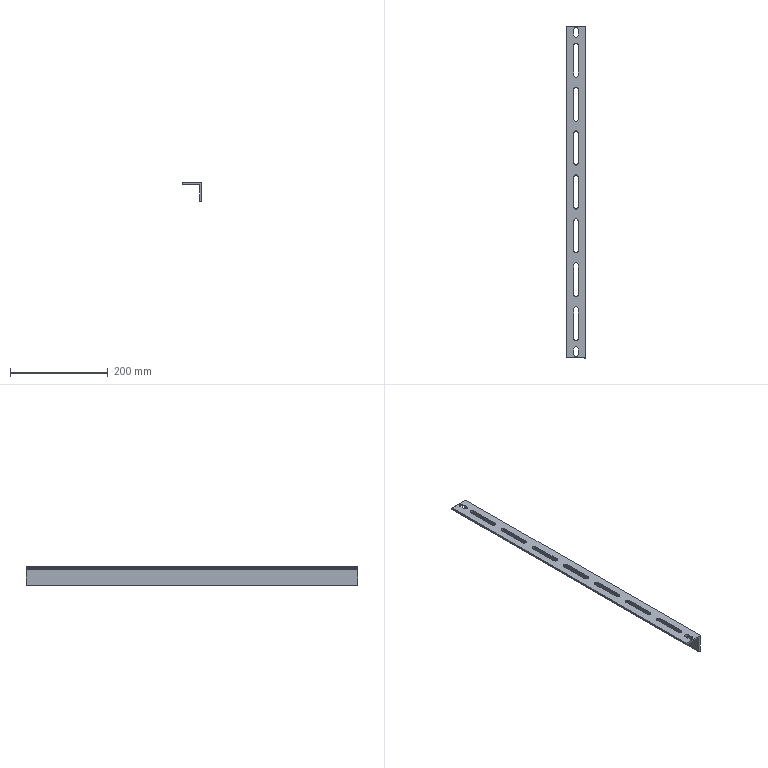Component | SolidWorks | BeamMountingAngleSteel-1 | 1 solid | 48 faces | box 40 x 680 x 40 mm | volume 189515 mm3 | plane 27 | cylinder 21 | commonest cylinder face diameters 9 x18 2.667 x2 7 x1
build123d program:
from build123d import *

# Parameters (mm, degrees)
BASE_DEPTH         = 680
CUT_EXTRUDE1_DEPTH = 5
CUT_EXTRUDE2_DEPTH = 5
CHAMFER1_SIZE      = 1


with BuildPart() as part:
    # Sketch1 → Base (new body)
    with BuildSketch(Plane.YZ):
        with BuildLine():
            Line((0, 40), (0, 0))
            Line((0, 0), (40, 0))
            Line((40, 0), (40, 2.667))
            ThreePointArc((40, 2.667), (39.609, 3.609), (38.667, 4))
            Line((38.667, 4), (7.5, 4))
            ThreePointArc((7.5, 4), (5.025, 5.025), (4, 7.5))
            Line((4, 7.5), (4, 38.667))
            ThreePointArc((4, 38.667), (3.609, 39.609), (2.667, 40))
            Line((2.667, 40), (0, 40))
        make_face()
    extrude(amount=BASE_DEPTH)

    # Sketch1_2 → Cut-Extrude1 (cut)
    with BuildSketch(Plane.XZ):
        with BuildLine():
            Line((672.5, 15.5), (661.5, 15.5))
            ThreePointArc((661.5, 15.5), (657, 20), (661.5, 24.5))
            Line((661.5, 24.5), (672.5, 24.5))
            ThreePointArc((672.5, 24.5), (677, 20), (672.5, 15.5))
        make_face()
        with BuildLine():
            Line((18.5, 15.5), (7.5, 15.5))
            ThreePointArc((7.5, 15.5), (3, 20), (7.5, 24.5))
            Line((7.5, 24.5), (18.5, 24.5))
            ThreePointArc((18.5, 24.5), (23, 20), (18.5, 15.5))
        make_face()
    extrude(amount=-CUT_EXTRUDE1_DEPTH, mode=Mode.SUBTRACT)

    # Sketch2 → Cut-Extrude2 (cut)
    with BuildSketch(Plane.XZ):
        with BuildLine():
            Line((370.5, 15.5), (309.5, 15.5))
            ThreePointArc((309.5, 15.5), (305, 20), (309.5, 24.5))
            Line((309.5, 24.5), (370.5, 24.5))
            ThreePointArc((370.5, 24.5), (375, 20), (370.5, 15.5))
        make_face()
        with BuildLine():
            Line((460.5, 15.5), (399.5, 15.5))
            ThreePointArc((399.5, 15.5), (395, 20), (399.5, 24.5))
            Line((399.5, 24.5), (460.5, 24.5))
            ThreePointArc((460.5, 24.5), (465, 20), (460.5, 15.5))
        make_face()
        with BuildLine():
            Line((550.5, 15.5), (489.5, 15.5))
            ThreePointArc((489.5, 15.5), (485, 20), (489.5, 24.5))
            Line((489.5, 24.5), (550.5, 24.5))
            ThreePointArc((550.5, 24.5), (555, 20), (550.5, 15.5))
        make_face()
        with BuildLine():
            Line((640.5, 15.5), (579.5, 15.5))
            ThreePointArc((579.5, 15.5), (575, 20), (579.5, 24.5))
            Line((579.5, 24.5), (640.5, 24.5))
            ThreePointArc((640.5, 24.5), (645, 20), (640.5, 15.5))
        make_face()
        with BuildLine():
            Line((280.5, 15.5), (219.5, 15.5))
            ThreePointArc((219.5, 15.5), (215, 20), (219.5, 24.5))
            Line((219.5, 24.5), (280.5, 24.5))
            ThreePointArc((280.5, 24.5), (285, 20), (280.5, 15.5))
        make_face()
        with BuildLine():
            Line((190.5, 15.5), (129.5, 15.5))
            ThreePointArc((129.5, 15.5), (125, 20), (129.5, 24.5))
            Line((129.5, 24.5), (190.5, 24.5))
            ThreePointArc((190.5, 24.5), (195, 20), (190.5, 15.5))
        make_face()
        with BuildLine():
            Line((100.5, 15.5), (39.5, 15.5))
            ThreePointArc((39.5, 15.5), (35, 20), (39.5, 24.5))
            Line((39.5, 24.5), (100.5, 24.5))
            ThreePointArc((100.5, 24.5), (105, 20), (100.5, 15.5))
        make_face()
    extrude(amount=-CUT_EXTRUDE2_DEPTH, mode=Mode.SUBTRACT)

    # Chamfer1
    chamfer1_edges = [part.edges().sort_by_distance(p)[0] for p in [
        (680, 0, 20),
    ]]
    chamfer(chamfer1_edges, length=CHAMFER1_SIZE)


solid = part.part

# Placed as in the assembly
solid = solid.moved(Location((-604.255, -194.605, 94), (-90, -90, 0)))